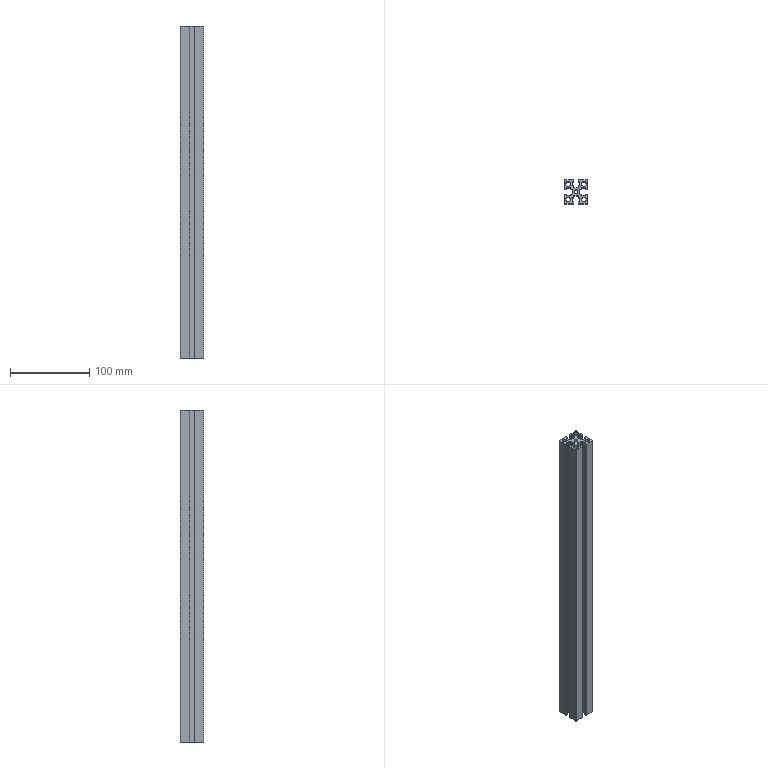Component | SolidWorks | XM-WST05-2007-1 | 1 solid | 116 faces | box 30 x 30 x 420 mm | volume 184972 mm3 | cylinder 62 | plane 54 | commonest cylinder face diameters 1 x48 6 x8 2 x4 5 x2
build123d program:
from build123d import *

# Parameters (mm, degrees)
SKETCH14_R               = 3
SKETCH14_R_2             = 2.5
STRUCTURAL_MEMBER1_DEPTH = 420


with BuildPart() as part:
    # Sketch14 → Structural Member1 (new body)
    with BuildSketch(Plane(origin=(0, 0, 0), x_dir=(-1, 0, 0), z_dir=(0, 1, 0))):
        with BuildLine():
            Line((3.15, 7), (3.15, 5.5))
            ThreePointArc((3.15, 5.5), (3.004, 5.146), (2.65, 5))
            Line((2.65, 5), (-2.65, 5))
            ThreePointArc((-2.65, 5), (-3.004, 5.146), (-3.15, 5.5))
            Line((-3.15, 5.5), (-3.15, 7))
            ThreePointArc((-3.15, 7), (-3.296, 7.354), (-3.65, 7.5))
            Line((-3.65, 7.5), (-4.5, 7.5))
            ThreePointArc((-4.5, 7.5), (-4.854, 7.646), (-5, 8))
            Line((-5, 8), (-5, 12))
            ThreePointArc((-5, 12), (-4.854, 12.354), (-4.5, 12.5))
            Line((-4.5, 12.5), (-3.65, 12.5))
            ThreePointArc((-3.65, 12.5), (-3.296, 12.646), (-3.15, 13))
            Line((-3.15, 13), (-3.15, 14.5))
            ThreePointArc((-3.15, 14.5), (-3.296, 14.854), (-3.65, 15))
            Line((-3.65, 15), (-14, 15))
            ThreePointArc((-14, 15), (-14.707, 14.707), (-15, 14))
            Line((-15, 14), (-15, 3.65))
            ThreePointArc((-15, 3.65), (-14.854, 3.296), (-14.5, 3.15))
            Line((-14.5, 3.15), (-13, 3.15))
            ThreePointArc((-13, 3.15), (-12.646, 3.296), (-12.5, 3.65))
            Line((-12.5, 3.65), (-12.5, 4.5))
            ThreePointArc((-12.5, 4.5), (-12.354, 4.854), (-12, 5))
            Line((-12, 5), (-8, 5))
            ThreePointArc((-8, 5), (-7.646, 4.854), (-7.5, 4.5))
            Line((-7.5, 4.5), (-7.5, 3.65))
            ThreePointArc((-7.5, 3.65), (-7.354, 3.296), (-7, 3.15))
            Line((-7, 3.15), (-5.5, 3.15))
            ThreePointArc((-5.5, 3.15), (-5.146, 3.004), (-5, 2.65))
            Line((-5, 2.65), (-5, -2.65))
            ThreePointArc((-5, -2.65), (-5.146, -3.004), (-5.5, -3.15))
            Line((-5.5, -3.15), (-7, -3.15))
            ThreePointArc((-7, -3.15), (-7.354, -3.296), (-7.5, -3.65))
            Line((-7.5, -3.65), (-7.5, -4.5))
            ThreePointArc((-7.5, -4.5), (-7.646, -4.854), (-8, -5))
            Line((-8, -5), (-12, -5))
            ThreePointArc((-12, -5), (-12.354, -4.854), (-12.5, -4.5))
            Line((-12.5, -4.5), (-12.5, -3.65))
            ThreePointArc((-12.5, -3.65), (-12.646, -3.296), (-13, -3.15))
            Line((-13, -3.15), (-14.5, -3.15))
            ThreePointArc((-14.5, -3.15), (-14.854, -3.296), (-15, -3.65))
            Line((-15, -3.65), (-15, -14))
            ThreePointArc((-15, -14), (-14.707, -14.707), (-14, -15))
            Line((-14, -15), (-3.65, -15))
            ThreePointArc((-3.65, -15), (-3.296, -14.854), (-3.15, -14.5))
            Line((-3.15, -14.5), (-3.15, -13))
            ThreePointArc((-3.15, -13), (-3.296, -12.646), (-3.65, -12.5))
            Line((-3.65, -12.5), (-4.5, -12.5))
            ThreePointArc((-4.5, -12.5), (-4.854, -12.354), (-5, -12))
            Line((-5, -12), (-5, -8))
            ThreePointArc((-5, -8), (-4.854, -7.646), (-4.5, -7.5))
            Line((-4.5, -7.5), (-3.65, -7.5))
            ThreePointArc((-3.65, -7.5), (-3.296, -7.354), (-3.15, -7))
            Line((-3.15, -7), (-3.15, -5.5))
            ThreePointArc((-3.15, -5.5), (-3.004, -5.146), (-2.65, -5))
            Line((-2.65, -5), (2.65, -5))
            ThreePointArc((2.65, -5), (3.004, -5.146), (3.15, -5.5))
            Line((3.15, -5.5), (3.15, -7))
            ThreePointArc((3.15, -7), (3.296, -7.354), (3.65, -7.5))
            Line((3.65, -7.5), (4.5, -7.5))
            ThreePointArc((4.5, -7.5), (4.854, -7.646), (5, -8))
            Line((5, -8), (5, -12))
            ThreePointArc((5, -12), (4.854, -12.354), (4.5, -12.5))
            Line((4.5, -12.5), (3.65, -12.5))
            ThreePointArc((3.65, -12.5), (3.296, -12.646), (3.15, -13))
            Line((3.15, -13), (3.15, -14.5))
            ThreePointArc((3.15, -14.5), (3.296, -14.854), (3.65, -15))
            Line((3.65, -15), (14, -15))
            ThreePointArc((14, -15), (14.707, -14.707), (15, -14))
            Line((15, -14), (15, -3.65))
            ThreePointArc((15, -3.65), (14.854, -3.296), (14.5, -3.15))
            Line((14.5, -3.15), (13, -3.15))
            ThreePointArc((13, -3.15), (12.646, -3.296), (12.5, -3.65))
            Line((12.5, -3.65), (12.5, -4.5))
            ThreePointArc((12.5, -4.5), (12.354, -4.854), (12, -5))
            Line((12, -5), (8, -5))
            ThreePointArc((8, -5), (7.646, -4.854), (7.5, -4.5))
            Line((7.5, -4.5), (7.5, -3.65))
            ThreePointArc((7.5, -3.65), (7.354, -3.296), (7, -3.15))
            Line((7, -3.15), (5.5, -3.15))
            ThreePointArc((5.5, -3.15), (5.146, -3.004), (5, -2.65))
            Line((5, -2.65), (5, 2.65))
            ThreePointArc((5, 2.65), (5.146, 3.004), (5.5, 3.15))
            Line((5.5, 3.15), (7, 3.15))
            ThreePointArc((7, 3.15), (7.354, 3.296), (7.5, 3.65))
            Line((7.5, 3.65), (7.5, 4.5))
            ThreePointArc((7.5, 4.5), (7.646, 4.854), (8, 5))
            Line((8, 5), (12, 5))
            ThreePointArc((12, 5), (12.354, 4.854), (12.5, 4.5))
            Line((12.5, 4.5), (12.5, 3.65))
            ThreePointArc((12.5, 3.65), (12.646, 3.296), (13, 3.15))
            Line((13, 3.15), (14.5, 3.15))
            ThreePointArc((14.5, 3.15), (14.854, 3.296), (15, 3.65))
            Line((15, 3.65), (15, 14))
            ThreePointArc((15, 14), (14.707, 14.707), (14, 15))
            Line((14, 15), (3.65, 15))
            ThreePointArc((3.65, 15), (3.296, 14.854), (3.15, 14.5))
            Line((3.15, 14.5), (3.15, 13))
            ThreePointArc((3.15, 13), (3.296, 12.646), (3.65, 12.5))
            Line((3.65, 12.5), (4.5, 12.5))
            ThreePointArc((4.5, 12.5), (4.854, 12.354), (5, 12))
            Line((5, 12), (5, 8))
            ThreePointArc((5, 8), (4.854, 7.646), (4.5, 7.5))
            Line((4.5, 7.5), (3.65, 7.5))
            ThreePointArc((3.65, 7.5), (3.296, 7.354), (3.15, 7))
        make_face()
        with Locations((10, 10)):
            Circle(SKETCH14_R, mode=Mode.SUBTRACT)
        with Locations((10, -10)):
            Circle(SKETCH14_R, mode=Mode.SUBTRACT)
        with Locations((-10, -10)):
            Circle(SKETCH14_R, mode=Mode.SUBTRACT)
        with Locations((-10, 10)):
            Circle(SKETCH14_R, mode=Mode.SUBTRACT)
        Circle(SKETCH14_R_2, mode=Mode.SUBTRACT)
    extrude(amount=STRUCTURAL_MEMBER1_DEPTH)


solid = part.part

# Placed as in the assembly
solid = solid.moved(Location((-154.071, 48.669, 100.899), (90, 0, 0)))